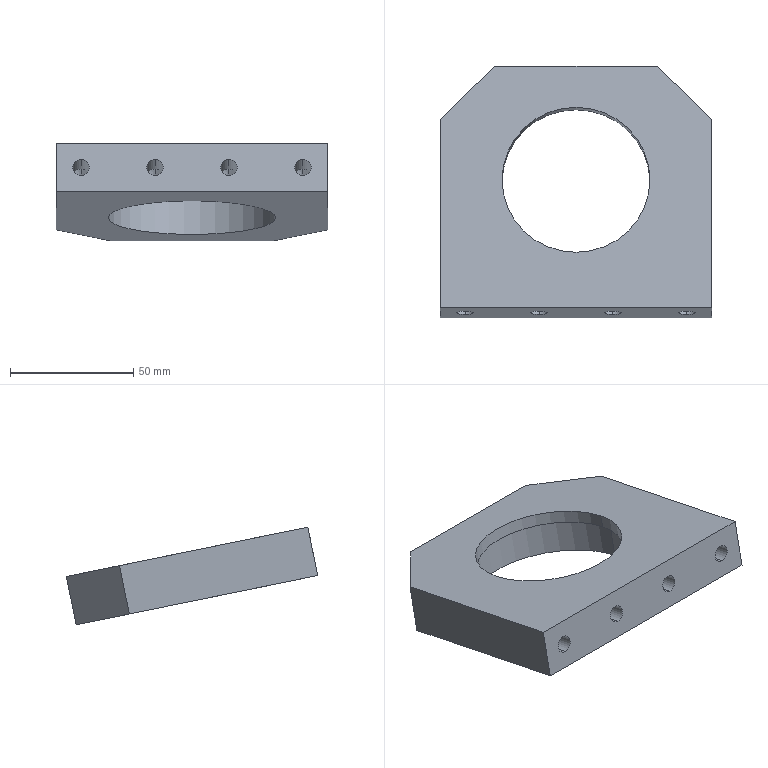Component | SolidWorks | JL001-04-01-006-1 | 1 solid | 29 faces | box 110 x 101.98 x 39.59 mm | volume 138740 mm3 | cylinder 12 | plane 9 | cone 8 | commonest cylinder face diameters 6.8 x8 60 x2 68 x2
build123d program:
from build123d import *

# Parameters (mm, degrees)
SKETCH1_W             = 110
SKETCH1_H             = 100
BOSS_EXTRUDE1_DEPTH   = 10
SKETCH2_R             = 34
CUT_EXTRUDE1_DEPTH    = 15
SKETCH3_R             = 30
CUT_EXTRUDE2_DEPTH    = 76.829
M8_TAPPED_HOLE1_D     = 6.8
M8_TAPPED_HOLE1_DEPTH = 19.75
M8_TAPPED_HOLE1_TIP   = 2.043
CHAMFER1_SIZE         = 22


with BuildPart() as part:
    # Sketch1 → Boss-Extrude1 (new, symmetric)
    with BuildSketch(Plane.XY):
        Rectangle(SKETCH1_W, SKETCH1_H)
    extrude(amount=BOSS_EXTRUDE1_DEPTH, both=True)

    # Sketch2 → Cut-Extrude1 (cut)
    with BuildSketch(Plane.XY.offset(10)):
        with Locations((0, 3)):
            Circle(SKETCH2_R)
    extrude(amount=-CUT_EXTRUDE1_DEPTH, mode=Mode.SUBTRACT)

    # Sketch3 → Cut-Extrude2 (cut, through all)
    with BuildSketch(Plane.XY.offset(-5)):
        with Locations((0, 3)):
            Circle(SKETCH3_R)
    extrude(amount=-CUT_EXTRUDE2_DEPTH, mode=Mode.SUBTRACT)

    # M8 Tapped Hole1
    with Locations(Plane(origin=(0, -50, 0), x_dir=(-1, 0, 0), z_dir=(0, -1, 0))):
        with Locations((45, 0), (15, 0), (-15, 0), (-45, 0)):
            Hole(M8_TAPPED_HOLE1_D / 2, depth=M8_TAPPED_HOLE1_DEPTH)
            with Locations((0, 0, -(M8_TAPPED_HOLE1_DEPTH + M8_TAPPED_HOLE1_TIP / 2))):  # 118° drill point
                Cone(0, M8_TAPPED_HOLE1_D / 2, M8_TAPPED_HOLE1_TIP, mode=Mode.SUBTRACT)

    # Chamfer1
    chamfer1_edges = [part.edges().sort_by_distance(p)[0] for p in [
        (-55, 50, 0),
        (55, 50, 0),
    ]]
    chamfer(chamfer1_edges, length=CHAMFER1_SIZE)


solid = part.part

# Placed as in the assembly
solid = solid.moved(Location((0, 191.783, 125.175), (168.465, 0, 180)))
STEP:
#1=COLOUR_RGB('',0.7922,0.8196,0.9333);
#2=FILL_AREA_STYLE_COLOUR('',#1);
#3=FILL_AREA_STYLE('',(#2));
#4=SURFACE_STYLE_FILL_AREA(#3);
#5=SURFACE_SIDE_STYLE('',(#4));
#6=SURFACE_STYLE_USAGE(.BOTH.,#5);
#7=PRESENTATION_STYLE_ASSIGNMENT((#6));
#8=CARTESIAN_POINT('',(1.772,6.357,5.035));
#9=VERTEX_POINT('',#8);
#10=CARTESIAN_POINT('',(1.772,6.41,5.297));
#11=VERTEX_POINT('',#10);
#12=CARTESIAN_POINT('',(1.772,6.384,5.166));
#13=DIRECTION('',(0.,-0.9798,0.2));
#14=DIRECTION('',(0.,0.2,0.9798));
#15=AXIS2_PLACEMENT_3D('',#12,#13,#14);
#16=CIRCLE('',#15,0.1339);
#17=EDGE_CURVE('',#9,#11,#16,.T.);
#18=ORIENTED_EDGE('',*,*,#17,.F.);
#19=CARTESIAN_POINT('',(1.772,5.595,5.191));
#20=VERTEX_POINT('',#19);
#21=CARTESIAN_POINT('',(1.772,5.595,5.191));
#22=DIRECTION('',(0.,-0.9798,0.2));
#23=VECTOR('',#22,39.37);
#24=LINE('',#21,#23);
#25=EDGE_CURVE('',#9,#20,#24,.T.);
#26=ORIENTED_EDGE('',*,*,#25,.T.);
#27=CARTESIAN_POINT('',(1.772,5.649,5.453));
#28=VERTEX_POINT('',#27);
#29=CARTESIAN_POINT('',(1.772,5.622,5.322));
#30=DIRECTION('',(0.,-0.9798,0.2));
#31=DIRECTION('',(0.,0.2,0.9798));
#32=AXIS2_PLACEMENT_3D('',#29,#30,#31);
#33=CIRCLE('',#32,0.1339);
#34=EDGE_CURVE('',#20,#28,#33,.T.);
#35=ORIENTED_EDGE('',*,*,#34,.T.);
#36=CARTESIAN_POINT('',(1.772,5.649,5.453));
#37=DIRECTION('',(0.,-0.9798,0.2));
#38=VECTOR('',#37,39.37);
#39=LINE('',#36,#38);
#40=EDGE_CURVE('',#11,#28,#39,.T.);
#41=ORIENTED_EDGE('',*,*,#40,.F.);
#42=EDGE_LOOP('',(#18,#26,#35,#41));
#43=FACE_OUTER_BOUND('',#42,.T.);
#44=CARTESIAN_POINT('',(1.772,5.622,5.322));
#45=DIRECTION('',(0.,-0.9798,0.2));
#46=DIRECTION('',(0.,0.2,0.9798));
#47=AXIS2_PLACEMENT_3D('',#44,#45,#46);
#48=CYLINDRICAL_SURFACE('',#47,0.1339);
#49=ADVANCED_FACE('',(#43),#48,.F.);
#50=CARTESIAN_POINT('',(1.772,6.462,5.15));
#51=VERTEX_POINT('',#50);
#52=CARTESIAN_POINT('',(1.772,6.41,5.297));
#53=DIRECTION('',(0.,-0.3332,0.9428));
#54=VECTOR('',#53,39.37);
#55=LINE('',#52,#54);
#56=EDGE_CURVE('',#51,#11,#55,.T.);
#57=ORIENTED_EDGE('',*,*,#56,.F.);
#58=CARTESIAN_POINT('',(1.772,6.357,5.035));
#59=DIRECTION('',(-0.,-0.676,-0.7369));
#60=VECTOR('',#59,39.37);
#61=LINE('',#58,#60);
#62=EDGE_CURVE('',#51,#9,#61,.T.);
#63=ORIENTED_EDGE('',*,*,#62,.T.);
#64=ORIENTED_EDGE('',*,*,#17,.T.);
#65=EDGE_LOOP('',(#57,#63,#64));
#66=FACE_OUTER_BOUND('',#65,.T.);
#67=CARTESIAN_POINT('',(1.772,6.384,5.166));
#68=DIRECTION('',(0.,-0.9798,0.2));
#69=DIRECTION('',(0.,0.2,0.9798));
#70=AXIS2_PLACEMENT_3D('',#67,#68,#69);
#71=CONICAL_SURFACE('',#70,0.1339,1.03);
#72=ADVANCED_FACE('',(#66),#71,.F.);
#73=CARTESIAN_POINT('',(0.5906,6.357,5.035));
#74=VERTEX_POINT('',#73);
#75=CARTESIAN_POINT('',(0.5906,6.41,5.297));
#76=VERTEX_POINT('',#75);
#77=CARTESIAN_POINT('',(0.5906,6.384,5.166));
#78=DIRECTION('',(0.,-0.9798,0.2));
#79=DIRECTION('',(0.,0.2,0.9798));
#80=AXIS2_PLACEMENT_3D('',#77,#78,#79);
#81=CIRCLE('',#80,0.1339);
#82=EDGE_CURVE('',#74,#76,#81,.T.);
#83=ORIENTED_EDGE('',*,*,#82,.F.);
#84=CARTESIAN_POINT('',(0.5906,5.595,5.191));
#85=VERTEX_POINT('',#84);
#86=CARTESIAN_POINT('',(0.5906,5.595,5.191));
#87=DIRECTION('',(0.,-0.9798,0.2));
#88=VECTOR('',#87,39.37);
#89=LINE('',#86,#88);
#90=EDGE_CURVE('',#74,#85,#89,.T.);
#91=ORIENTED_EDGE('',*,*,#90,.T.);
#92=CARTESIAN_POINT('',(0.5906,5.649,5.453));
#93=VERTEX_POINT('',#92);
#94=CARTESIAN_POINT('',(0.5906,5.622,5.322));
#95=DIRECTION('',(0.,-0.9798,0.2));
#96=DIRECTION('',(0.,0.2,0.9798));
#97=AXIS2_PLACEMENT_3D('',#94,#95,#96);
#98=CIRCLE('',#97,0.1339);
#99=EDGE_CURVE('',#85,#93,#98,.T.);
#100=ORIENTED_EDGE('',*,*,#99,.T.);
#101=CARTESIAN_POINT('',(0.5906,5.649,5.453));
#102=DIRECTION('',(0.,-0.9798,0.2));
#103=VECTOR('',#102,39.37);
#104=LINE('',#101,#103);
#105=EDGE_CURVE('',#76,#93,#104,.T.);
#106=ORIENTED_EDGE('',*,*,#105,.F.);
#107=EDGE_LOOP('',(#83,#91,#100,#106));
#108=FACE_OUTER_BOUND('',#107,.T.);
#109=CARTESIAN_POINT('',(0.5906,5.622,5.322));
#110=DIRECTION('',(0.,-0.9798,0.2));
#111=DIRECTION('',(0.,0.2,0.9798));
#112=AXIS2_PLACEMENT_3D('',#109,#110,#111);
#113=CYLINDRICAL_SURFACE('',#112,0.1339);
#114=ADVANCED_FACE('',(#108),#113,.F.);
#115=CARTESIAN_POINT('',(0.5906,6.462,5.15));
#116=VERTEX_POINT('',#115);
#117=CARTESIAN_POINT('',(0.5906,6.41,5.297));
#118=DIRECTION('',(0.,-0.3332,0.9428));
#119=VECTOR('',#118,39.37);
#120=LINE('',#117,#119);
#121=EDGE_CURVE('',#116,#76,#120,.T.);
#122=ORIENTED_EDGE('',*,*,#121,.F.);
#123=CARTESIAN_POINT('',(0.5906,6.357,5.035));
#124=DIRECTION('',(-0.,-0.676,-0.7369));
#125=VECTOR('',#124,39.37);
#126=LINE('',#123,#125);
#127=EDGE_CURVE('',#116,#74,#126,.T.);
#128=ORIENTED_EDGE('',*,*,#127,.T.);
#129=ORIENTED_EDGE('',*,*,#82,.T.);
#130=EDGE_LOOP('',(#122,#128,#129));
#131=FACE_OUTER_BOUND('',#130,.T.);
#132=CARTESIAN_POINT('',(0.5906,6.384,5.166));
#133=DIRECTION('',(0.,-0.9798,0.2));
#134=DIRECTION('',(0.,0.2,0.9798));
#135=AXIS2_PLACEMENT_3D('',#132,#133,#134);
#136=CONICAL_SURFACE('',#135,0.1339,1.03);
#137=ADVANCED_FACE('',(#131),#136,.F.);
#138=CARTESIAN_POINT('',(-0.5906,6.357,5.035));
#139=VERTEX_POINT('',#138);
#140=CARTESIAN_POINT('',(-0.5906,6.41,5.297));
#141=VERTEX_POINT('',#140);
#142=CARTESIAN_POINT('',(-0.5906,6.384,5.166));
#143=DIRECTION('',(0.,-0.9798,0.2));
#144=DIRECTION('',(0.,0.2,0.9798));
#145=AXIS2_PLACEMENT_3D('',#142,#143,#144);
#146=CIRCLE('',#145,0.1339);
#147=EDGE_CURVE('',#139,#141,#146,.T.);
#148=ORIENTED_EDGE('',*,*,#147,.F.);
#149=CARTESIAN_POINT('',(-0.5906,5.595,5.191));
#150=VERTEX_POINT('',#149);
#151=CARTESIAN_POINT('',(-0.5906,5.595,5.191));
#152=DIRECTION('',(0.,-0.9798,0.2));
#153=VECTOR('',#152,39.37);
#154=LINE('',#151,#153);
#155=EDGE_CURVE('',#139,#150,#154,.T.);
#156=ORIENTED_EDGE('',*,*,#155,.T.);
#157=CARTESIAN_POINT('',(-0.5906,5.649,5.453));
#158=VERTEX_POINT('',#157);
#159=CARTESIAN_POINT('',(-0.5906,5.622,5.322));
#160=DIRECTION('',(0.,-0.9798,0.2));
#161=DIRECTION('',(0.,0.2,0.9798));
#162=AXIS2_PLACEMENT_3D('',#159,#160,#161);
#163=CIRCLE('',#162,0.1339);
#164=EDGE_CURVE('',#150,#158,#163,.T.);
#165=ORIENTED_EDGE('',*,*,#164,.T.);
#166=CARTESIAN_POINT('',(-0.5906,5.649,5.453));
#167=DIRECTION('',(0.,-0.9798,0.2));
#168=VECTOR('',#167,39.37);
#169=LINE('',#166,#168);
#170=EDGE_CURVE('',#141,#158,#169,.T.);
#171=ORIENTED_EDGE('',*,*,#170,.F.);
#172=EDGE_LOOP('',(#148,#156,#165,#171));
#173=FACE_OUTER_BOUND('',#172,.T.);
#174=CARTESIAN_POINT('',(-0.5906,5.622,5.322));
#175=DIRECTION('',(0.,-0.9798,0.2));
#176=DIRECTION('',(0.,0.2,0.9798));
#177=AXIS2_PLACEMENT_3D('',#174,#175,#176);
#178=CYLINDRICAL_SURFACE('',#177,0.1339);
#179=ADVANCED_FACE('',(#173),#178,.F.);
#180=CARTESIAN_POINT('',(-0.5906,6.462,5.15));
#181=VERTEX_POINT('',#180);
#182=CARTESIAN_POINT('',(-0.5906,6.41,5.297));
#183=DIRECTION('',(0.,-0.3332,0.9428));
#184=VECTOR('',#183,39.37);
#185=LINE('',#182,#184);
#186=EDGE_CURVE('',#181,#141,#185,.T.);
#187=ORIENTED_EDGE('',*,*,#186,.F.);
#188=CARTESIAN_POINT('',(-0.5906,6.357,5.035));
#189=DIRECTION('',(-0.,-0.676,-0.7369));
#190=VECTOR('',#189,39.37);
#191=LINE('',#188,#190);
#192=EDGE_CURVE('',#181,#139,#191,.T.);
#193=ORIENTED_EDGE('',*,*,#192,.T.);
#194=ORIENTED_EDGE('',*,*,#147,.T.);
#195=EDGE_LOOP('',(#187,#193,#194));
#196=FACE_OUTER_BOUND('',#195,.T.);
#197=CARTESIAN_POINT('',(-0.5906,6.384,5.166));
#198=DIRECTION('',(0.,-0.9798,0.2));
#199=DIRECTION('',(0.,0.2,0.9798));
#200=AXIS2_PLACEMENT_3D('',#197,#198,#199);
#201=CONICAL_SURFACE('',#200,0.1339,1.03);
#202=ADVANCED_FACE('',(#196),#201,.F.);
#203=CARTESIAN_POINT('',(-1.772,6.357,5.035));
#204=VERTEX_POINT('',#203);
#205=CARTESIAN_POINT('',(-1.772,6.41,5.297));
#206=VERTEX_POINT('',#205);
#207=CARTESIAN_POINT('',(-1.772,6.384,5.166));
#208=DIRECTION('',(0.,-0.9798,0.2));
#209=DIRECTION('',(0.,0.2,0.9798));
#210=AXIS2_PLACEMENT_3D('',#207,#208,#209);
#211=CIRCLE('',#210,0.1339);
#212=EDGE_CURVE('',#204,#206,#211,.T.);
#213=ORIENTED_EDGE('',*,*,#212,.F.);
#214=CARTESIAN_POINT('',(-1.772,5.595,5.191));
#215=VERTEX_POINT('',#214);
#216=CARTESIAN_POINT('',(-1.772,5.595,5.191));
#217=DIRECTION('',(0.,-0.9798,0.2));
#218=VECTOR('',#217,39.37);
#219=LINE('',#216,#218);
#220=EDGE_CURVE('',#204,#215,#219,.T.);
#221=ORIENTED_EDGE('',*,*,#220,.T.);
#222=CARTESIAN_POINT('',(-1.772,5.649,5.453));
#223=VERTEX_POINT('',#222);
#224=CARTESIAN_POINT('',(-1.772,5.622,5.322));
#225=DIRECTION('',(0.,-0.9798,0.2));
#226=DIRECTION('',(0.,0.2,0.9798));
#227=AXIS2_PLACEMENT_3D('',#224,#225,#226);
#228=CIRCLE('',#227,0.1339);
#229=EDGE_CURVE('',#215,#223,#228,.T.);
#230=ORIENTED_EDGE('',*,*,#229,.T.);
#231=CARTESIAN_POINT('',(-1.772,5.649,5.453));
#232=DIRECTION('',(0.,-0.9798,0.2));
#233=VECTOR('',#232,39.37);
#234=LINE('',#231,#233);
#235=EDGE_CURVE('',#206,#223,#234,.T.);
#236=ORIENTED_EDGE('',*,*,#235,.F.);
#237=EDGE_LOOP('',(#213,#221,#230,#236));
#238=FACE_OUTER_BOUND('',#237,.T.);
#239=CARTESIAN_POINT('',(-1.772,5.622,5.322));
#240=DIRECTION('',(0.,-0.9798,0.2));
#241=DIRECTION('',(0.,0.2,0.9798));
#242=AXIS2_PLACEMENT_3D('',#239,#240,#241);
#243=CYLINDRICAL_SURFACE('',#242,0.1339);
#244=ADVANCED_FACE('',(#238),#243,.F.);
#245=CARTESIAN_POINT('',(-1.772,6.462,5.15));
#246=VERTEX_POINT('',#245);
#247=CARTESIAN_POINT('',(-1.772,6.41,5.297));
#248=DIRECTION('',(0.,-0.3332,0.9428));
#249=VECTOR('',#248,39.37);
#250=LINE('',#247,#249);
#251=EDGE_CURVE('',#246,#206,#250,.T.);
#252=ORIENTED_EDGE('',*,*,#251,.F.);
#253=CARTESIAN_POINT('',(-1.772,6.357,5.035));
#254=DIRECTION('',(-0.,-0.676,-0.7369));
#255=VECTOR('',#254,39.37);
#256=LINE('',#253,#255);
#257=EDGE_CURVE('',#246,#204,#256,.T.);
#258=ORIENTED_EDGE('',*,*,#257,.T.);
#259=ORIENTED_EDGE('',*,*,#212,.T.);
#260=EDGE_LOOP('',(#252,#258,#259));
#261=FACE_OUTER_BOUND('',#260,.T.);
#262=CARTESIAN_POINT('',(-1.772,6.384,5.166));
#263=DIRECTION('',(0.,-0.9798,0.2));
#264=DIRECTION('',(0.,0.2,0.9798));
#265=AXIS2_PLACEMENT_3D('',#262,#263,#264);
#266=CONICAL_SURFACE('',#265,0.1339,1.03);
#267=ADVANCED_FACE('',(#261),#266,.F.);
#268=CARTESIAN_POINT('',(1.181,7.745,5.29));
#269=VERTEX_POINT('',#268);
#270=CARTESIAN_POINT('',(-1.181,7.745,5.29));
#271=VERTEX_POINT('',#270);
#272=CARTESIAN_POINT('',(-0.,7.745,5.29));
#273=DIRECTION('',(-0.,-0.2,-0.9798));
#274=DIRECTION('',(-1.,0.,0.));
#275=AXIS2_PLACEMENT_3D('',#272,#273,#274);
#276=CIRCLE('',#275,1.181);
#277=EDGE_CURVE('',#269,#271,#276,.T.);
#278=ORIENTED_EDGE('',*,*,#277,.F.);
#279=CARTESIAN_POINT('',(1.181,7.706,5.097));
#280=VERTEX_POINT('',#279);
#281=CARTESIAN_POINT('',(1.181,7.745,5.29));
#282=DIRECTION('',(-0.,-0.2,-0.9798));
#283=VECTOR('',#282,39.37);
#284=LINE('',#281,#283);
#285=EDGE_CURVE('',#269,#280,#284,.T.);
#286=ORIENTED_EDGE('',*,*,#285,.T.);
#287=CARTESIAN_POINT('',(-1.181,7.706,5.097));
#288=VERTEX_POINT('',#287);
#289=CARTESIAN_POINT('',(-0.,7.706,5.097));
#290=DIRECTION('',(-0.,-0.2,-0.9798));
#291=DIRECTION('',(-1.,0.,0.));
#292=AXIS2_PLACEMENT_3D('',#289,#290,#291);
#293=CIRCLE('',#292,1.181);
#294=EDGE_CURVE('',#280,#288,#293,.T.);
#295=ORIENTED_EDGE('',*,*,#294,.T.);
#296=CARTESIAN_POINT('',(-1.181,7.745,5.29));
#297=DIRECTION('',(-0.,-0.2,-0.9798));
#298=VECTOR('',#297,39.37);
#299=LINE('',#296,#298);
#300=EDGE_CURVE('',#271,#288,#299,.T.);
#301=ORIENTED_EDGE('',*,*,#300,.F.);
#302=EDGE_LOOP('',(#278,#286,#295,#301));
#303=FACE_OUTER_BOUND('',#302,.T.);
#304=CARTESIAN_POINT('',(-0.,7.745,5.29));
#305=DIRECTION('',(-0.,-0.2,-0.9798));
#306=DIRECTION('',(-1.,0.,0.));
#307=AXIS2_PLACEMENT_3D('',#304,#305,#306);
#308=CYLINDRICAL_SURFACE('',#307,1.181);
#309=ADVANCED_FACE('',(#303),#308,.F.);
#310=CARTESIAN_POINT('',(1.339,7.706,5.097));
#311=VERTEX_POINT('',#310);
#312=CARTESIAN_POINT('',(-1.339,7.706,5.097));
#313=VERTEX_POINT('',#312);
#314=CARTESIAN_POINT('',(-0.,7.706,5.097));
#315=DIRECTION('',(-0.,-0.2,-0.9798));
#316=DIRECTION('',(-1.,0.,0.));
#317=AXIS2_PLACEMENT_3D('',#314,#315,#316);
#318=CIRCLE('',#317,1.339);
#319=EDGE_CURVE('',#311,#313,#318,.T.);
#320=ORIENTED_EDGE('',*,*,#319,.F.);
#321=CARTESIAN_POINT('',(1.339,7.587,4.519));
#322=VERTEX_POINT('',#321);
#323=CARTESIAN_POINT('',(1.339,7.706,5.097));
#324=DIRECTION('',(-0.,-0.2,-0.9798));
#325=VECTOR('',#324,39.37);
#326=LINE('',#323,#325);
#327=EDGE_CURVE('',#311,#322,#326,.T.);
#328=ORIENTED_EDGE('',*,*,#327,.T.);
#329=CARTESIAN_POINT('',(-1.339,7.587,4.519));
#330=VERTEX_POINT('',#329);
#331=CARTESIAN_POINT('',(-0.,7.587,4.519));
#332=DIRECTION('',(-0.,-0.2,-0.9798));
#333=DIRECTION('',(-1.,0.,0.));
#334=AXIS2_PLACEMENT_3D('',#331,#332,#333);
#335=CIRCLE('',#334,1.339);
#336=EDGE_CURVE('',#322,#330,#335,.T.);
#337=ORIENTED_EDGE('',*,*,#336,.T.);
#338=CARTESIAN_POINT('',(-1.339,7.706,5.097));
#339=DIRECTION('',(-0.,-0.2,-0.9798));
#340=VECTOR('',#339,39.37);
#341=LINE('',#338,#340);
#342=EDGE_CURVE('',#313,#330,#341,.T.);
#343=ORIENTED_EDGE('',*,*,#342,.F.);
#344=EDGE_LOOP('',(#320,#328,#337,#343));
#345=FACE_OUTER_BOUND('',#344,.T.);
#346=CARTESIAN_POINT('',(-0.,7.706,5.097));
#347=DIRECTION('',(-0.,-0.2,-0.9798));
#348=DIRECTION('',(-1.,0.,0.));
#349=AXIS2_PLACEMENT_3D('',#346,#347,#348);
#350=CYLINDRICAL_SURFACE('',#349,1.339);
#351=ADVANCED_FACE('',(#345),#350,.F.);
#352=CARTESIAN_POINT('',(-2.165,5.7,5.708));
#353=VERTEX_POINT('',#352);
#354=CARTESIAN_POINT('',(-2.165,8.709,5.093));
#355=VERTEX_POINT('',#354);
#356=CARTESIAN_POINT('',(-2.165,9.558,4.92));
#357=DIRECTION('',(0.,0.9798,-0.2));
#358=VECTOR('',#357,39.37);
#359=LINE('',#356,#358);
#360=EDGE_CURVE('',#353,#355,#359,.T.);
#361=ORIENTED_EDGE('',*,*,#360,.T.);
#362=CARTESIAN_POINT('',(-2.165,8.552,4.322));
#363=VERTEX_POINT('',#362);
#364=CARTESIAN_POINT('',(-2.165,8.552,4.322));
#365=DIRECTION('',(-0.,-0.2,-0.9798));
#366=VECTOR('',#365,39.37);
#367=LINE('',#364,#366);
#368=EDGE_CURVE('',#355,#363,#367,.T.);
#369=ORIENTED_EDGE('',*,*,#368,.T.);
#370=CARTESIAN_POINT('',(-2.165,5.543,4.936));
#371=VERTEX_POINT('',#370);
#372=CARTESIAN_POINT('',(-2.165,9.401,4.149));
#373=DIRECTION('',(0.,0.9798,-0.2));
#374=VECTOR('',#373,39.37);
#375=LINE('',#372,#374);
#376=EDGE_CURVE('',#371,#363,#375,.T.);
#377=ORIENTED_EDGE('',*,*,#376,.F.);
#378=CARTESIAN_POINT('',(-2.165,5.543,4.936));
#379=DIRECTION('',(0.,0.2,0.9798));
#380=VECTOR('',#379,39.37);
#381=LINE('',#378,#380);
#382=EDGE_CURVE('',#371,#353,#381,.T.);
#383=ORIENTED_EDGE('',*,*,#382,.T.);
#384=EDGE_LOOP('',(#361,#369,#377,#383));
#385=FACE_OUTER_BOUND('',#384,.T.);
#386=CARTESIAN_POINT('',(-2.165,9.401,4.149));
#387=DIRECTION('',(1.,-0.,0.));
#388=DIRECTION('',(-0.,-0.9798,0.2));
#389=AXIS2_PLACEMENT_3D('',#386,#387,#388);
#390=PLANE('',#389);
#391=ADVANCED_FACE('',(#385),#390,.F.);
#392=CARTESIAN_POINT('',(-1.299,9.558,4.92));
#393=VERTEX_POINT('',#392);
#394=CARTESIAN_POINT('',(1.299,9.558,4.92));
#395=VERTEX_POINT('',#394);
#396=CARTESIAN_POINT('',(2.165,9.558,4.92));
#397=DIRECTION('',(1.,-0.,-0.));
#398=VECTOR('',#397,39.37);
#399=LINE('',#396,#398);
#400=EDGE_CURVE('',#393,#395,#399,.T.);
#401=ORIENTED_EDGE('',*,*,#400,.T.);
#402=CARTESIAN_POINT('',(1.299,9.401,4.149));
#403=VERTEX_POINT('',#402);
#404=CARTESIAN_POINT('',(1.299,9.401,4.149));
#405=DIRECTION('',(-0.,-0.2,-0.9798));
#406=VECTOR('',#405,39.37);
#407=LINE('',#404,#406);
#408=EDGE_CURVE('',#395,#403,#407,.T.);
#409=ORIENTED_EDGE('',*,*,#408,.T.);
#410=CARTESIAN_POINT('',(-1.299,9.401,4.149));
#411=VERTEX_POINT('',#410);
#412=CARTESIAN_POINT('',(2.165,9.401,4.149));
#413=DIRECTION('',(1.,-0.,-0.));
#414=VECTOR('',#413,39.37);
#415=LINE('',#412,#414);
#416=EDGE_CURVE('',#411,#403,#415,.T.);
#417=ORIENTED_EDGE('',*,*,#416,.F.);
#418=CARTESIAN_POINT('',(-1.299,9.401,4.149));
#419=DIRECTION('',(0.,0.2,0.9798));
#420=VECTOR('',#419,39.37);
#421=LINE('',#418,#420);
#422=EDGE_CURVE('',#411,#393,#421,.T.);
#423=ORIENTED_EDGE('',*,*,#422,.T.);
#424=EDGE_LOOP('',(#401,#409,#417,#423));
#425=FACE_OUTER_BOUND('',#424,.T.);
#426=CARTESIAN_POINT('',(2.165,9.401,4.149));
#427=DIRECTION('',(0.,-0.9798,0.2));
#428=DIRECTION('',(0.,0.2,0.9798));
#429=AXIS2_PLACEMENT_3D('',#426,#427,#428);
#430=PLANE('',#429);
#431=ADVANCED_FACE('',(#425),#430,.F.);
#432=CARTESIAN_POINT('',(2.165,8.552,4.322));
#433=VERTEX_POINT('',#432);
#434=CARTESIAN_POINT('',(2.165,5.543,4.936));
#435=VERTEX_POINT('',#434);
#436=CARTESIAN_POINT('',(2.165,9.401,4.149));
#437=DIRECTION('',(-0.,-0.9798,0.2));
#438=VECTOR('',#437,39.37);
#439=LINE('',#436,#438);
#440=EDGE_CURVE('',#433,#435,#439,.T.);
#441=ORIENTED_EDGE('',*,*,#440,.F.);
#442=CARTESIAN_POINT('',(2.165,8.709,5.093));
#443=VERTEX_POINT('',#442);
#444=CARTESIAN_POINT('',(2.165,8.552,4.322));
#445=DIRECTION('',(0.,0.2,0.9798));
#446=VECTOR('',#445,39.37);
#447=LINE('',#444,#446);
#448=EDGE_CURVE('',#433,#443,#447,.T.);
#449=ORIENTED_EDGE('',*,*,#448,.T.);
#450=CARTESIAN_POINT('',(2.165,5.7,5.708));
#451=VERTEX_POINT('',#450);
#452=CARTESIAN_POINT('',(2.165,9.558,4.92));
#453=DIRECTION('',(-0.,-0.9798,0.2));
#454=VECTOR('',#453,39.37);
#455=LINE('',#452,#454);
#456=EDGE_CURVE('',#443,#451,#455,.T.);
#457=ORIENTED_EDGE('',*,*,#456,.T.);
#458=CARTESIAN_POINT('',(2.165,5.543,4.936));
#459=DIRECTION('',(0.,0.2,0.9798));
#460=VECTOR('',#459,39.37);
#461=LINE('',#458,#460);
#462=EDGE_CURVE('',#435,#451,#461,.T.);
#463=ORIENTED_EDGE('',*,*,#462,.F.);
#464=EDGE_LOOP('',(#441,#449,#457,#463));
#465=FACE_OUTER_BOUND('',#464,.T.);
#466=CARTESIAN_POINT('',(2.165,9.401,4.149));
#467=DIRECTION('',(-1.,0.,-0.));
#468=DIRECTION('',(0.,0.9798,-0.2));
#469=AXIS2_PLACEMENT_3D('',#466,#467,#468);
#470=PLANE('',#469);
#471=ADVANCED_FACE('',(#465),#470,.F.);
#472=CARTESIAN_POINT('',(1.772,5.622,5.322));
#473=DIRECTION('',(0.,-0.9798,0.2));
#474=DIRECTION('',(0.,0.2,0.9798));
#475=AXIS2_PLACEMENT_3D('',#472,#473,#474);
#476=CIRCLE('',#475,0.1339);
#477=EDGE_CURVE('',#28,#20,#476,.T.);
#478=ORIENTED_EDGE('',*,*,#477,.F.);
#479=ORIENTED_EDGE('',*,*,#34,.F.);
#480=EDGE_LOOP('',(#478,#479));
#481=FACE_BOUND('',#480,.T.);
#482=CARTESIAN_POINT('',(0.5906,5.622,5.322));
#483=DIRECTION('',(0.,-0.9798,0.2));
#484=DIRECTION('',(0.,0.2,0.9798));
#485=AXIS2_PLACEMENT_3D('',#482,#483,#484);
#486=CIRCLE('',#485,0.1339);
#487=EDGE_CURVE('',#93,#85,#486,.T.);
#488=ORIENTED_EDGE('',*,*,#487,.F.);
#489=ORIENTED_EDGE('',*,*,#99,.F.);
#490=EDGE_LOOP('',(#488,#489));
#491=FACE_BOUND('',#490,.T.);
#492=CARTESIAN_POINT('',(-0.5906,5.622,5.322));
#493=DIRECTION('',(0.,-0.9798,0.2));
#494=DIRECTION('',(0.,0.2,0.9798));
#495=AXIS2_PLACEMENT_3D('',#492,#493,#494);
#496=CIRCLE('',#495,0.1339);
#497=EDGE_CURVE('',#158,#150,#496,.T.);
#498=ORIENTED_EDGE('',*,*,#497,.F.);
#499=ORIENTED_EDGE('',*,*,#164,.F.);
#500=EDGE_LOOP('',(#498,#499));
#501=FACE_BOUND('',#500,.T.);
#502=CARTESIAN_POINT('',(-1.772,5.622,5.322));
#503=DIRECTION('',(0.,-0.9798,0.2));
#504=DIRECTION('',(0.,0.2,0.9798));
#505=AXIS2_PLACEMENT_3D('',#502,#503,#504);
#506=CIRCLE('',#505,0.1339);
#507=EDGE_CURVE('',#223,#215,#506,.T.);
#508=ORIENTED_EDGE('',*,*,#507,.F.);
#509=ORIENTED_EDGE('',*,*,#229,.F.);
#510=EDGE_LOOP('',(#508,#509));
#511=FACE_BOUND('',#510,.T.);
#512=CARTESIAN_POINT('',(2.165,5.7,5.708));
#513=DIRECTION('',(-1.,0.,0.));
#514=VECTOR('',#513,39.37);
#515=LINE('',#512,#514);
#516=EDGE_CURVE('',#451,#353,#515,.T.);
#517=ORIENTED_EDGE('',*,*,#516,.T.);
#518=ORIENTED_EDGE('',*,*,#382,.F.);
#519=CARTESIAN_POINT('',(2.165,5.543,4.936));
#520=DIRECTION('',(-1.,0.,0.));
#521=VECTOR('',#520,39.37);
#522=LINE('',#519,#521);
#523=EDGE_CURVE('',#435,#371,#522,.T.);
#524=ORIENTED_EDGE('',*,*,#523,.F.);
#525=ORIENTED_EDGE('',*,*,#462,.T.);
#526=EDGE_LOOP('',(#517,#518,#524,#525));
#527=FACE_OUTER_BOUND('',#526,.T.);
#528=CARTESIAN_POINT('',(2.165,5.543,4.936));
#529=DIRECTION('',(-0.,0.9798,-0.2));
#530=DIRECTION('',(-0.,-0.2,-0.9798));
#531=AXIS2_PLACEMENT_3D('',#528,#529,#530);
#532=PLANE('',#531);
#533=ADVANCED_FACE('',(#481,#491,#501,#511,#527),#532,.F.);
#534=CARTESIAN_POINT('',(-0.,7.587,4.519));
#535=DIRECTION('',(-0.,-0.2,-0.9798));
#536=DIRECTION('',(-1.,0.,0.));
#537=AXIS2_PLACEMENT_3D('',#534,#535,#536);
#538=CIRCLE('',#537,1.339);
#539=EDGE_CURVE('',#330,#322,#538,.T.);
#540=ORIENTED_EDGE('',*,*,#539,.F.);
#541=ORIENTED_EDGE('',*,*,#336,.F.);
#542=EDGE_LOOP('',(#540,#541));
#543=FACE_BOUND('',#542,.T.);
#544=ORIENTED_EDGE('',*,*,#416,.T.);
#545=CARTESIAN_POINT('',(1.634,9.073,4.216));
#546=DIRECTION('',(0.7071,-0.6928,0.1414));
#547=VECTOR('',#546,39.37);
#548=LINE('',#545,#547);
#549=EDGE_CURVE('',#403,#433,#548,.T.);
#550=ORIENTED_EDGE('',*,*,#549,.T.);
#551=ORIENTED_EDGE('',*,*,#440,.T.);
#552=ORIENTED_EDGE('',*,*,#523,.T.);
#553=ORIENTED_EDGE('',*,*,#376,.T.);
#554=CARTESIAN_POINT('',(-1.634,9.073,4.216));
#555=DIRECTION('',(0.7071,0.6928,-0.1414));
#556=VECTOR('',#555,39.37);
#557=LINE('',#554,#556);
#558=EDGE_CURVE('',#363,#411,#557,.T.);
#559=ORIENTED_EDGE('',*,*,#558,.T.);
#560=EDGE_LOOP('',(#544,#550,#551,#552,#553,#559));
#561=FACE_OUTER_BOUND('',#560,.T.);
#562=CARTESIAN_POINT('',(-0.,7.472,4.542));
#563=DIRECTION('',(-0.,-0.2,-0.9798));
#564=DIRECTION('',(-1.,0.,0.));
#565=AXIS2_PLACEMENT_3D('',#562,#563,#564);
#566=PLANE('',#565);
#567=ADVANCED_FACE('',(#543,#561),#566,.T.);
#568=CARTESIAN_POINT('',(-0.,7.745,5.29));
#569=DIRECTION('',(-0.,-0.2,-0.9798));
#570=DIRECTION('',(-1.,0.,0.));
#571=AXIS2_PLACEMENT_3D('',#568,#569,#570);
#572=CIRCLE('',#571,1.181);
#573=EDGE_CURVE('',#271,#269,#572,.T.);
#574=ORIENTED_EDGE('',*,*,#573,.T.);
#575=ORIENTED_EDGE('',*,*,#277,.T.);
#576=EDGE_LOOP('',(#574,#575));
#577=FACE_BOUND('',#576,.T.);
#578=ORIENTED_EDGE('',*,*,#456,.F.);
#579=CARTESIAN_POINT('',(2.165,8.709,5.093));
#580=DIRECTION('',(-0.7071,0.6928,-0.1414));
#581=VECTOR('',#580,39.37);
#582=LINE('',#579,#581);
#583=EDGE_CURVE('',#443,#395,#582,.T.);
#584=ORIENTED_EDGE('',*,*,#583,.T.);
#585=ORIENTED_EDGE('',*,*,#400,.F.);
#586=CARTESIAN_POINT('',(-1.299,9.558,4.92));
#587=DIRECTION('',(-0.7071,-0.6928,0.1414));
#588=VECTOR('',#587,39.37);
#589=LINE('',#586,#588);
#590=EDGE_CURVE('',#393,#355,#589,.T.);
#591=ORIENTED_EDGE('',*,*,#590,.T.);
#592=ORIENTED_EDGE('',*,*,#360,.F.);
#593=ORIENTED_EDGE('',*,*,#516,.F.);
#594=EDGE_LOOP('',(#578,#584,#585,#591,#592,#593));
#595=FACE_OUTER_BOUND('',#594,.T.);
#596=CARTESIAN_POINT('',(-0.,7.629,5.314));
#597=DIRECTION('',(-0.,-0.2,-0.9798));
#598=DIRECTION('',(-1.,0.,0.));
#599=AXIS2_PLACEMENT_3D('',#596,#597,#598);
#600=PLANE('',#599);
#601=ADVANCED_FACE('',(#577,#595),#600,.F.);
#602=ORIENTED_EDGE('',*,*,#327,.F.);
#603=CARTESIAN_POINT('',(-0.,7.706,5.097));
#604=DIRECTION('',(-0.,-0.2,-0.9798));
#605=DIRECTION('',(-1.,0.,0.));
#606=AXIS2_PLACEMENT_3D('',#603,#604,#605);
#607=CIRCLE('',#606,1.339);
#608=EDGE_CURVE('',#313,#311,#607,.T.);
#609=ORIENTED_EDGE('',*,*,#608,.F.);
#610=ORIENTED_EDGE('',*,*,#342,.T.);
#611=ORIENTED_EDGE('',*,*,#539,.T.);
#612=EDGE_LOOP('',(#602,#609,#610,#611));
#613=FACE_OUTER_BOUND('',#612,.T.);
#614=CARTESIAN_POINT('',(-0.,7.706,5.097));
#615=DIRECTION('',(-0.,-0.2,-0.9798));
#616=DIRECTION('',(-1.,0.,0.));
#617=AXIS2_PLACEMENT_3D('',#614,#615,#616);
#618=CYLINDRICAL_SURFACE('',#617,1.339);
#619=ADVANCED_FACE('',(#613),#618,.F.);
#620=CARTESIAN_POINT('',(-0.,7.706,5.097));
#621=DIRECTION('',(-0.,-0.2,-0.9798));
#622=DIRECTION('',(-1.,0.,0.));
#623=AXIS2_PLACEMENT_3D('',#620,#621,#622);
#624=CIRCLE('',#623,1.181);
#625=EDGE_CURVE('',#288,#280,#624,.T.);
#626=ORIENTED_EDGE('',*,*,#625,.F.);
#627=ORIENTED_EDGE('',*,*,#294,.F.);
#628=EDGE_LOOP('',(#626,#627));
#629=FACE_BOUND('',#628,.T.);
#630=ORIENTED_EDGE('',*,*,#608,.T.);
#631=ORIENTED_EDGE('',*,*,#319,.T.);
#632=EDGE_LOOP('',(#630,#631));
#633=FACE_OUTER_BOUND('',#632,.T.);
#634=CARTESIAN_POINT('',(-0.,7.706,5.097));
#635=DIRECTION('',(-0.,-0.2,-0.9798));
#636=DIRECTION('',(-1.,0.,0.));
#637=AXIS2_PLACEMENT_3D('',#634,#635,#636);
#638=PLANE('',#637);
#639=ADVANCED_FACE('',(#629,#633),#638,.T.);
#640=ORIENTED_EDGE('',*,*,#285,.F.);
#641=ORIENTED_EDGE('',*,*,#573,.F.);
#642=ORIENTED_EDGE('',*,*,#300,.T.);
#643=ORIENTED_EDGE('',*,*,#625,.T.);
#644=EDGE_LOOP('',(#640,#641,#642,#643));
#645=FACE_OUTER_BOUND('',#644,.T.);
#646=CARTESIAN_POINT('',(-0.,7.745,5.29));
#647=DIRECTION('',(-0.,-0.2,-0.9798));
#648=DIRECTION('',(-1.,0.,0.));
#649=AXIS2_PLACEMENT_3D('',#646,#647,#648);
#650=CYLINDRICAL_SURFACE('',#649,1.181);
#651=ADVANCED_FACE('',(#645),#650,.F.);
#652=ORIENTED_EDGE('',*,*,#257,.F.);
#653=ORIENTED_EDGE('',*,*,#251,.T.);
#654=CARTESIAN_POINT('',(-1.772,6.384,5.166));
#655=DIRECTION('',(0.,-0.9798,0.2));
#656=DIRECTION('',(0.,0.2,0.9798));
#657=AXIS2_PLACEMENT_3D('',#654,#655,#656);
#658=CIRCLE('',#657,0.1339);
#659=EDGE_CURVE('',#206,#204,#658,.T.);
#660=ORIENTED_EDGE('',*,*,#659,.T.);
#661=EDGE_LOOP('',(#652,#653,#660));
#662=FACE_OUTER_BOUND('',#661,.T.);
#663=CARTESIAN_POINT('',(-1.772,6.384,5.166));
#664=DIRECTION('',(0.,-0.9798,0.2));
#665=DIRECTION('',(0.,0.2,0.9798));
#666=AXIS2_PLACEMENT_3D('',#663,#664,#665);
#667=CONICAL_SURFACE('',#666,0.1339,1.03);
#668=ADVANCED_FACE('',(#662),#667,.F.);
#669=ORIENTED_EDGE('',*,*,#220,.F.);
#670=ORIENTED_EDGE('',*,*,#659,.F.);
#671=ORIENTED_EDGE('',*,*,#235,.T.);
#672=ORIENTED_EDGE('',*,*,#507,.T.);
#673=EDGE_LOOP('',(#669,#670,#671,#672));
#674=FACE_OUTER_BOUND('',#673,.T.);
#675=CARTESIAN_POINT('',(-1.772,5.622,5.322));
#676=DIRECTION('',(0.,-0.9798,0.2));
#677=DIRECTION('',(0.,0.2,0.9798));
#678=AXIS2_PLACEMENT_3D('',#675,#676,#677);
#679=CYLINDRICAL_SURFACE('',#678,0.1339);
#680=ADVANCED_FACE('',(#674),#679,.F.);
#681=ORIENTED_EDGE('',*,*,#192,.F.);
#682=ORIENTED_EDGE('',*,*,#186,.T.);
#683=CARTESIAN_POINT('',(-0.5906,6.384,5.166));
#684=DIRECTION('',(0.,-0.9798,0.2));
#685=DIRECTION('',(0.,0.2,0.9798));
#686=AXIS2_PLACEMENT_3D('',#683,#684,#685);
#687=CIRCLE('',#686,0.1339);
#688=EDGE_CURVE('',#141,#139,#687,.T.);
#689=ORIENTED_EDGE('',*,*,#688,.T.);
#690=EDGE_LOOP('',(#681,#682,#689));
#691=FACE_OUTER_BOUND('',#690,.T.);
#692=CARTESIAN_POINT('',(-0.5906,6.384,5.166));
#693=DIRECTION('',(0.,-0.9798,0.2));
#694=DIRECTION('',(0.,0.2,0.9798));
#695=AXIS2_PLACEMENT_3D('',#692,#693,#694);
#696=CONICAL_SURFACE('',#695,0.1339,1.03);
#697=ADVANCED_FACE('',(#691),#696,.F.);
#698=ORIENTED_EDGE('',*,*,#155,.F.);
#699=ORIENTED_EDGE('',*,*,#688,.F.);
#700=ORIENTED_EDGE('',*,*,#170,.T.);
#701=ORIENTED_EDGE('',*,*,#497,.T.);
#702=EDGE_LOOP('',(#698,#699,#700,#701));
#703=FACE_OUTER_BOUND('',#702,.T.);
#704=CARTESIAN_POINT('',(-0.5906,5.622,5.322));
#705=DIRECTION('',(0.,-0.9798,0.2));
#706=DIRECTION('',(0.,0.2,0.9798));
#707=AXIS2_PLACEMENT_3D('',#704,#705,#706);
#708=CYLINDRICAL_SURFACE('',#707,0.1339);
#709=ADVANCED_FACE('',(#703),#708,.F.);
#710=ORIENTED_EDGE('',*,*,#127,.F.);
#711=ORIENTED_EDGE('',*,*,#121,.T.);
#712=CARTESIAN_POINT('',(0.5906,6.384,5.166));
#713=DIRECTION('',(0.,-0.9798,0.2));
#714=DIRECTION('',(0.,0.2,0.9798));
#715=AXIS2_PLACEMENT_3D('',#712,#713,#714);
#716=CIRCLE('',#715,0.1339);
#717=EDGE_CURVE('',#76,#74,#716,.T.);
#718=ORIENTED_EDGE('',*,*,#717,.T.);
#719=EDGE_LOOP('',(#710,#711,#718));
#720=FACE_OUTER_BOUND('',#719,.T.);
#721=CARTESIAN_POINT('',(0.5906,6.384,5.166));
#722=DIRECTION('',(0.,-0.9798,0.2));
#723=DIRECTION('',(0.,0.2,0.9798));
#724=AXIS2_PLACEMENT_3D('',#721,#722,#723);
#725=CONICAL_SURFACE('',#724,0.1339,1.03);
#726=ADVANCED_FACE('',(#720),#725,.F.);
#727=ORIENTED_EDGE('',*,*,#90,.F.);
#728=ORIENTED_EDGE('',*,*,#717,.F.);
#729=ORIENTED_EDGE('',*,*,#105,.T.);
#730=ORIENTED_EDGE('',*,*,#487,.T.);
#731=EDGE_LOOP('',(#727,#728,#729,#730));
#732=FACE_OUTER_BOUND('',#731,.T.);
#733=CARTESIAN_POINT('',(0.5906,5.622,5.322));
#734=DIRECTION('',(0.,-0.9798,0.2));
#735=DIRECTION('',(0.,0.2,0.9798));
#736=AXIS2_PLACEMENT_3D('',#733,#734,#735);
#737=CYLINDRICAL_SURFACE('',#736,0.1339);
#738=ADVANCED_FACE('',(#732),#737,.F.);
#739=ORIENTED_EDGE('',*,*,#62,.F.);
#740=ORIENTED_EDGE('',*,*,#56,.T.);
#741=CARTESIAN_POINT('',(1.772,6.384,5.166));
#742=DIRECTION('',(0.,-0.9798,0.2));
#743=DIRECTION('',(0.,0.2,0.9798));
#744=AXIS2_PLACEMENT_3D('',#741,#742,#743);
#745=CIRCLE('',#744,0.1339);
#746=EDGE_CURVE('',#11,#9,#745,.T.);
#747=ORIENTED_EDGE('',*,*,#746,.T.);
#748=EDGE_LOOP('',(#739,#740,#747));
#749=FACE_OUTER_BOUND('',#748,.T.);
#750=CARTESIAN_POINT('',(1.772,6.384,5.166));
#751=DIRECTION('',(0.,-0.9798,0.2));
#752=DIRECTION('',(0.,0.2,0.9798));
#753=AXIS2_PLACEMENT_3D('',#750,#751,#752);
#754=CONICAL_SURFACE('',#753,0.1339,1.03);
#755=ADVANCED_FACE('',(#749),#754,.F.);
#756=ORIENTED_EDGE('',*,*,#25,.F.);
#757=ORIENTED_EDGE('',*,*,#746,.F.);
#758=ORIENTED_EDGE('',*,*,#40,.T.);
#759=ORIENTED_EDGE('',*,*,#477,.T.);
#760=EDGE_LOOP('',(#756,#757,#758,#759));
#761=FACE_OUTER_BOUND('',#760,.T.);
#762=CARTESIAN_POINT('',(1.772,5.622,5.322));
#763=DIRECTION('',(0.,-0.9798,0.2));
#764=DIRECTION('',(0.,0.2,0.9798));
#765=AXIS2_PLACEMENT_3D('',#762,#763,#764);
#766=CYLINDRICAL_SURFACE('',#765,0.1339);
#767=ADVANCED_FACE('',(#761),#766,.F.);
#768=ORIENTED_EDGE('',*,*,#549,.F.);
#769=ORIENTED_EDGE('',*,*,#408,.F.);
#770=ORIENTED_EDGE('',*,*,#583,.F.);
#771=ORIENTED_EDGE('',*,*,#448,.F.);
#772=EDGE_LOOP('',(#768,#769,#770,#771));
#773=FACE_OUTER_BOUND('',#772,.T.);
#774=CARTESIAN_POINT('',(2.165,8.552,4.322));
#775=DIRECTION('',(-0.7071,-0.6928,0.1414));
#776=DIRECTION('',(0.,0.2,0.9798));
#777=AXIS2_PLACEMENT_3D('',#774,#775,#776);
#778=PLANE('',#777);
#779=ADVANCED_FACE('',(#773),#778,.F.);
#780=ORIENTED_EDGE('',*,*,#558,.F.);
#781=ORIENTED_EDGE('',*,*,#368,.F.);
#782=ORIENTED_EDGE('',*,*,#590,.F.);
#783=ORIENTED_EDGE('',*,*,#422,.F.);
#784=EDGE_LOOP('',(#780,#781,#782,#783));
#785=FACE_OUTER_BOUND('',#784,.T.);
#786=CARTESIAN_POINT('',(-1.299,9.401,4.149));
#787=DIRECTION('',(0.7071,-0.6928,0.1414));
#788=DIRECTION('',(0.,0.2,0.9798));
#789=AXIS2_PLACEMENT_3D('',#786,#787,#788);
#790=PLANE('',#789);
#791=ADVANCED_FACE('',(#785),#790,.F.);
#792=CLOSED_SHELL('',(#49,#72,#114,#137,#179,#202,#244,#267,#309,#351,#391,#431,#471,#533,#567,#601,#619,#639,#651,#668,#680,#697,#709,#726,#738,#755,#767,#779,#791));
#793=MANIFOLD_SOLID_BREP('',#792);
#794=STYLED_ITEM('',(#7),#793);
#795=PRESENTATION_LAYER_ASSIGNMENT('','',(#794));
#796=(LENGTH_UNIT()NAMED_UNIT(*)SI_UNIT($,.METRE.));
#797=LENGTH_MEASURE_WITH_UNIT(LENGTH_MEASURE(0.0254),#796);
#798=DIMENSIONAL_EXPONENTS(1.,0.,0.,0.,0.,0.,0.);
#799=(CONVERSION_BASED_UNIT('',#797)LENGTH_UNIT()NAMED_UNIT(#798));
#800=UNCERTAINTY_MEASURE_WITH_UNIT(LENGTH_MEASURE(0.00001),#799,'','');
#801=(NAMED_UNIT(*)PLANE_ANGLE_UNIT()SI_UNIT($,.RADIAN.));
#802=(NAMED_UNIT(*)SI_UNIT($,.STERADIAN.)SOLID_ANGLE_UNIT());
#803=(GEOMETRIC_REPRESENTATION_CONTEXT(3)GLOBAL_UNCERTAINTY_ASSIGNED_CONTEXT((#800))GLOBAL_UNIT_ASSIGNED_CONTEXT((#799,#801,#802))REPRESENTATION_CONTEXT('',''));
#804=MECHANICAL_DESIGN_GEOMETRIC_PRESENTATION_REPRESENTATION('',(#794),#803);
#805=CARTESIAN_POINT('',(0.,0.,0.));
#806=DIRECTION('',(0.,0.,1.));
#807=DIRECTION('',(1.,0.,0.));
#808=AXIS2_PLACEMENT_3D('',#805,#806,#807);
#809=(LENGTH_UNIT()NAMED_UNIT(*)SI_UNIT($,.METRE.));
#810=LENGTH_MEASURE_WITH_UNIT(LENGTH_MEASURE(0.0254),#809);
#811=DIMENSIONAL_EXPONENTS(1.,0.,0.,0.,0.,0.,0.);
#812=(CONVERSION_BASED_UNIT('',#810)LENGTH_UNIT()NAMED_UNIT(#811));
#813=UNCERTAINTY_MEASURE_WITH_UNIT(LENGTH_MEASURE(0.00001),#812,'','');
#814=(NAMED_UNIT(*)PLANE_ANGLE_UNIT()SI_UNIT($,.RADIAN.));
#815=(NAMED_UNIT(*)SI_UNIT($,.STERADIAN.)SOLID_ANGLE_UNIT());
#816=(GEOMETRIC_REPRESENTATION_CONTEXT(3)GLOBAL_UNCERTAINTY_ASSIGNED_CONTEXT((#813))GLOBAL_UNIT_ASSIGNED_CONTEXT((#812,#814,#815))REPRESENTATION_CONTEXT('',''));
#817=ADVANCED_BREP_SHAPE_REPRESENTATION('',(#793,#808),#816);